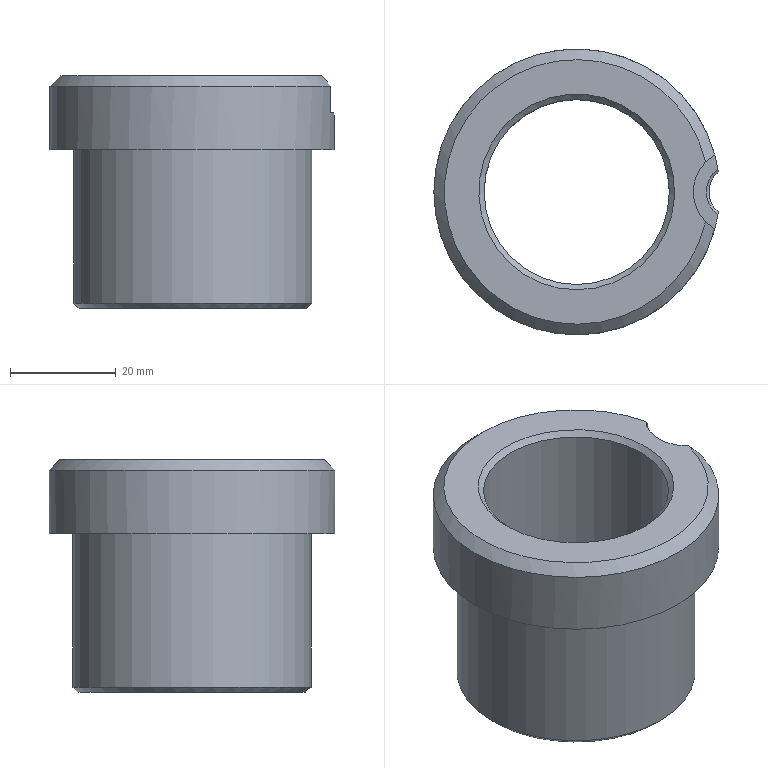Component | NX | DRILL_BUSH | 1 solid | 14 faces | box 53.73 x 54 x 44 mm | volume 36540 mm3 | cylinder 5 | cone 5 | plane 4 | commonest cylinder face diameters 45 x1 54 x1 35 x1 10 x1 16 x1
STEP:
#1=CARTESIAN_POINT('',(0.,0.,0.));
#2=DIRECTION('',(0.,0.,1.));
#3=DIRECTION('',(1.,0.,0.));
#4=AXIS2_PLACEMENT_3D('',#1,#2,#3);
#5=CARTESIAN_POINT('',(-37.,21.5,64.));
#6=VERTEX_POINT('',#5);
#7=CARTESIAN_POINT('',(-37.,-0.,64.));
#8=DIRECTION('',(0.,0.,-1.));
#9=DIRECTION('',(0.,1.,0.));
#10=AXIS2_PLACEMENT_3D('',#7,#8,#9);
#11=CIRCLE('',#10,21.5);
#12=CARTESIAN_POINT('',(-37.,-0.,64.));
#13=DIRECTION('',(0.,0.,-1.));
#14=DIRECTION('',(0.,1.,0.));
#15=AXIS2_PLACEMENT_3D('',#12,#13,#14);
#16=PLANE('',#15);
#17=CARTESIAN_POINT('',(0.,0.));
#18=DIRECTION('',(1.,0.));
#19=AXIS2_PLACEMENT_2D('',#17,#18);
#20=CIRCLE('',#19,21.5);
#21=(GEOMETRIC_REPRESENTATION_CONTEXT(2)PARAMETRIC_REPRESENTATION_CONTEXT()REPRESENTATION_CONTEXT('',''));
#22=DEFINITIONAL_REPRESENTATION('',(#20),#21);
#23=PCURVE('',#16,#22);
#24=CARTESIAN_POINT('',(-37.,-0.,65.));
#25=DIRECTION('',(0.,0.,1.));
#26=DIRECTION('',(0.,-1.,0.));
#27=AXIS2_PLACEMENT_3D('',#24,#25,#26);
#28=CONICAL_SURFACE('',#27,22.5,0.7854);
#29=CARTESIAN_POINT('',(9.425,-1.));
#30=DIRECTION('',(-1.,0.));
#31=VECTOR('',#30,1.);
#32=LINE('',#29,#31);
#33=(GEOMETRIC_REPRESENTATION_CONTEXT(2)PARAMETRIC_REPRESENTATION_CONTEXT()REPRESENTATION_CONTEXT('',''));
#34=DEFINITIONAL_REPRESENTATION('',(#32),#33);
#35=PCURVE('',#28,#34);
#36=SURFACE_CURVE('',#11,(#23,#35),.PCURVE_S1.);
#37=EDGE_CURVE('',#6,#6,#36,.T.);
#38=ORIENTED_EDGE('',*,*,#37,.T.);
#39=EDGE_LOOP('',(#38));
#40=FACE_BOUND('',#39,.T.);
#41=CARTESIAN_POINT('',(-37.,18.5,64.));
#42=VERTEX_POINT('',#41);
#43=CARTESIAN_POINT('',(-37.,-0.,64.));
#44=DIRECTION('',(0.,0.,1.));
#45=DIRECTION('',(0.,1.,0.));
#46=AXIS2_PLACEMENT_3D('',#43,#44,#45);
#47=CIRCLE('',#46,18.5);
#48=CARTESIAN_POINT('',(18.5,0.));
#49=CARTESIAN_POINT('',(18.5,-32.043));
#50=CARTESIAN_POINT('',(-9.25,-16.021));
#51=CARTESIAN_POINT('',(-37.,-0.));
#52=CARTESIAN_POINT('',(-9.25,16.021));
#53=CARTESIAN_POINT('',(18.5,32.043));
#54=CARTESIAN_POINT('',(18.5,0.));
#55=(BOUNDED_CURVE()B_SPLINE_CURVE(2,(#48,#49,#50,#51,#52,#53,#54),.UNSPECIFIED.,.T.,.F.)B_SPLINE_CURVE_WITH_KNOTS((1,2,2,2,2,1),(-2.094,0.,2.094,4.189,6.283,8.378),.UNSPECIFIED.)CURVE()GEOMETRIC_REPRESENTATION_ITEM()RATIONAL_B_SPLINE_CURVE((1.,0.5,1.,0.5,1.,0.5,1.))REPRESENTATION_ITEM(''));
#56=(GEOMETRIC_REPRESENTATION_CONTEXT(2)PARAMETRIC_REPRESENTATION_CONTEXT()REPRESENTATION_CONTEXT('',''));
#57=DEFINITIONAL_REPRESENTATION('',(#55),#56);
#58=PCURVE('',#16,#57);
#59=CARTESIAN_POINT('',(-37.,-0.,65.));
#60=DIRECTION('',(0.,0.,-1.));
#61=DIRECTION('',(0.,1.,0.));
#62=AXIS2_PLACEMENT_3D('',#59,#60,#61);
#63=CONICAL_SURFACE('',#62,17.5,0.7854);
#64=CARTESIAN_POINT('',(6.283,1.));
#65=DIRECTION('',(-1.,0.));
#66=VECTOR('',#65,1.);
#67=LINE('',#64,#66);
#68=(GEOMETRIC_REPRESENTATION_CONTEXT(2)PARAMETRIC_REPRESENTATION_CONTEXT()REPRESENTATION_CONTEXT('',''));
#69=DEFINITIONAL_REPRESENTATION('',(#67),#68);
#70=PCURVE('',#63,#69);
#71=SURFACE_CURVE('',#47,(#58,#70),.PCURVE_S1.);
#72=EDGE_CURVE('',#42,#42,#71,.T.);
#73=ORIENTED_EDGE('',*,*,#72,.T.);
#74=EDGE_LOOP('',(#73));
#75=FACE_BOUND('',#74,.T.);
#76=ADVANCED_FACE('',(#40,#75),#16,.T.);
#77=CARTESIAN_POINT('',(-37.,22.5,65.));
#78=VERTEX_POINT('',#77);
#79=CARTESIAN_POINT('',(-37.,-0.,65.));
#80=DIRECTION('',(0.,0.,1.));
#81=DIRECTION('',(0.,1.,0.));
#82=AXIS2_PLACEMENT_3D('',#79,#80,#81);
#83=CIRCLE('',#82,22.5);
#84=CARTESIAN_POINT('',(-37.,-0.,64.));
#85=DIRECTION('',(0.,0.,1.));
#86=DIRECTION('',(0.,-1.,0.));
#87=AXIS2_PLACEMENT_3D('',#84,#85,#86);
#88=CYLINDRICAL_SURFACE('',#87,22.5);
#89=CARTESIAN_POINT('',(3.142,1.));
#90=DIRECTION('',(1.,0.));
#91=VECTOR('',#90,1.);
#92=LINE('',#89,#91);
#93=(GEOMETRIC_REPRESENTATION_CONTEXT(2)PARAMETRIC_REPRESENTATION_CONTEXT()REPRESENTATION_CONTEXT('',''));
#94=DEFINITIONAL_REPRESENTATION('',(#92),#93);
#95=PCURVE('',#88,#94);
#96=CARTESIAN_POINT('',(3.142,0.));
#97=DIRECTION('',(1.,0.));
#98=VECTOR('',#97,1.);
#99=LINE('',#96,#98);
#100=(GEOMETRIC_REPRESENTATION_CONTEXT(2)PARAMETRIC_REPRESENTATION_CONTEXT()REPRESENTATION_CONTEXT('',''));
#101=DEFINITIONAL_REPRESENTATION('',(#99),#100);
#102=PCURVE('',#28,#101);
#103=SURFACE_CURVE('',#83,(#95,#102),.PCURVE_S1.);
#104=EDGE_CURVE('',#78,#78,#103,.T.);
#105=ORIENTED_EDGE('',*,*,#104,.T.);
#106=CARTESIAN_POINT('',(-37.,22.5,94.));
#107=VERTEX_POINT('',#106);
#108=CARTESIAN_POINT('',(-37.,22.5,65.));
#109=CARTESIAN_POINT('',(-37.,22.5,94.));
#110=B_SPLINE_CURVE_WITH_KNOTS('',1,(#108,#109),.UNSPECIFIED.,.F.,.F.,(2,2),(1.,30.),.PIECEWISE_BEZIER_KNOTS.);
#111=CARTESIAN_POINT('',(9.425,0.));
#112=DIRECTION('',(0.,1.));
#113=VECTOR('',#112,1.);
#114=LINE('',#111,#113);
#115=(GEOMETRIC_REPRESENTATION_CONTEXT(2)PARAMETRIC_REPRESENTATION_CONTEXT()REPRESENTATION_CONTEXT('',''));
#116=DEFINITIONAL_REPRESENTATION('',(#114),#115);
#117=PCURVE('',#88,#116);
#118=CARTESIAN_POINT('',(3.142,0.));
#119=DIRECTION('',(0.,1.));
#120=VECTOR('',#119,1.);
#121=LINE('',#118,#120);
#122=(GEOMETRIC_REPRESENTATION_CONTEXT(2)PARAMETRIC_REPRESENTATION_CONTEXT()REPRESENTATION_CONTEXT('',''));
#123=DEFINITIONAL_REPRESENTATION('',(#121),#122);
#124=PCURVE('',#88,#123);
#125=SEAM_CURVE('',#110,(#117,#124),.PCURVE_S1.);
#126=EDGE_CURVE('',#78,#107,#125,.T.);
#127=ORIENTED_EDGE('',*,*,#126,.T.);
#128=CARTESIAN_POINT('',(-37.,-0.,94.));
#129=DIRECTION('',(0.,0.,1.));
#130=DIRECTION('',(0.,1.,0.));
#131=AXIS2_PLACEMENT_3D('',#128,#129,#130);
#132=CIRCLE('',#131,22.5);
#133=CARTESIAN_POINT('',(3.142,30.));
#134=DIRECTION('',(1.,0.));
#135=VECTOR('',#134,1.);
#136=LINE('',#133,#135);
#137=(GEOMETRIC_REPRESENTATION_CONTEXT(2)PARAMETRIC_REPRESENTATION_CONTEXT()REPRESENTATION_CONTEXT('',''));
#138=DEFINITIONAL_REPRESENTATION('',(#136),#137);
#139=PCURVE('',#88,#138);
#140=CARTESIAN_POINT('',(-37.,-0.,94.));
#141=DIRECTION('',(0.,0.,-1.));
#142=DIRECTION('',(0.,1.,0.));
#143=AXIS2_PLACEMENT_3D('',#140,#141,#142);
#144=PLANE('',#143);
#145=CARTESIAN_POINT('',(22.5,0.));
#146=CARTESIAN_POINT('',(22.5,-38.971));
#147=CARTESIAN_POINT('',(-11.25,-19.486));
#148=CARTESIAN_POINT('',(-45.,-0.));
#149=CARTESIAN_POINT('',(-11.25,19.486));
#150=CARTESIAN_POINT('',(22.5,38.971));
#151=CARTESIAN_POINT('',(22.5,0.));
#152=(BOUNDED_CURVE()B_SPLINE_CURVE(2,(#145,#146,#147,#148,#149,#150,#151),.UNSPECIFIED.,.T.,.F.)B_SPLINE_CURVE_WITH_KNOTS((1,2,2,2,2,1),(-2.094,0.,2.094,4.189,6.283,8.378),.UNSPECIFIED.)CURVE()GEOMETRIC_REPRESENTATION_ITEM()RATIONAL_B_SPLINE_CURVE((1.,0.5,1.,0.5,1.,0.5,1.))REPRESENTATION_ITEM(''));
#153=(GEOMETRIC_REPRESENTATION_CONTEXT(2)PARAMETRIC_REPRESENTATION_CONTEXT()REPRESENTATION_CONTEXT('',''));
#154=DEFINITIONAL_REPRESENTATION('',(#152),#153);
#155=PCURVE('',#144,#154);
#156=SURFACE_CURVE('',#132,(#139,#155),.PCURVE_S1.);
#157=EDGE_CURVE('',#107,#107,#156,.T.);
#158=ORIENTED_EDGE('',*,*,#157,.F.);
#159=ORIENTED_EDGE('',*,*,#126,.F.);
#160=EDGE_LOOP('',(#105,#127,#158,#159));
#161=FACE_BOUND('',#160,.T.);
#162=ADVANCED_FACE('',(#161),#88,.T.);
#163=CARTESIAN_POINT('',(-37.,-18.5,108.));
#164=VERTEX_POINT('',#163);
#165=CARTESIAN_POINT('',(-37.,-0.,108.));
#166=DIRECTION('',(0.,0.,-1.));
#167=DIRECTION('',(0.,-1.,0.));
#168=AXIS2_PLACEMENT_3D('',#165,#166,#167);
#169=CIRCLE('',#168,18.5);
#170=CARTESIAN_POINT('',(-37.,-0.,108.));
#171=DIRECTION('',(0.,0.,1.));
#172=DIRECTION('',(0.,-1.,0.));
#173=AXIS2_PLACEMENT_3D('',#170,#171,#172);
#174=PLANE('',#173);
#175=CARTESIAN_POINT('',(18.5,0.));
#176=CARTESIAN_POINT('',(18.5,-32.043));
#177=CARTESIAN_POINT('',(-9.25,-16.021));
#178=CARTESIAN_POINT('',(-37.,-0.));
#179=CARTESIAN_POINT('',(-9.25,16.021));
#180=CARTESIAN_POINT('',(18.5,32.043));
#181=CARTESIAN_POINT('',(18.5,0.));
#182=(BOUNDED_CURVE()B_SPLINE_CURVE(2,(#175,#176,#177,#178,#179,#180,#181),.UNSPECIFIED.,.T.,.F.)B_SPLINE_CURVE_WITH_KNOTS((1,2,2,2,2,1),(-2.094,0.,2.094,4.189,6.283,8.378),.UNSPECIFIED.)CURVE()GEOMETRIC_REPRESENTATION_ITEM()RATIONAL_B_SPLINE_CURVE((1.,0.5,1.,0.5,1.,0.5,1.))REPRESENTATION_ITEM(''));
#183=(GEOMETRIC_REPRESENTATION_CONTEXT(2)PARAMETRIC_REPRESENTATION_CONTEXT()REPRESENTATION_CONTEXT('',''));
#184=DEFINITIONAL_REPRESENTATION('',(#182),#183);
#185=PCURVE('',#174,#184);
#186=CARTESIAN_POINT('',(-37.,-0.,108.));
#187=DIRECTION('',(0.,0.,1.));
#188=DIRECTION('',(0.,-1.,0.));
#189=AXIS2_PLACEMENT_3D('',#186,#187,#188);
#190=CONICAL_SURFACE('',#189,18.5,0.7854);
#191=CARTESIAN_POINT('',(6.283,0.));
#192=DIRECTION('',(-1.,0.));
#193=VECTOR('',#192,1.);
#194=LINE('',#191,#193);
#195=(GEOMETRIC_REPRESENTATION_CONTEXT(2)PARAMETRIC_REPRESENTATION_CONTEXT()REPRESENTATION_CONTEXT('',''));
#196=DEFINITIONAL_REPRESENTATION('',(#194),#195);
#197=PCURVE('',#190,#196);
#198=SURFACE_CURVE('',#169,(#185,#197),.PCURVE_S1.);
#199=EDGE_CURVE('',#164,#164,#198,.T.);
#200=ORIENTED_EDGE('',*,*,#199,.T.);
#201=EDGE_LOOP('',(#200));
#202=FACE_BOUND('',#201,.T.);
#203=CARTESIAN_POINT('',(-12.65,-5.664,108.));
#204=VERTEX_POINT('',#203);
#205=CARTESIAN_POINT('',(-12.65,5.664,108.));
#206=VERTEX_POINT('',#205);
#207=CARTESIAN_POINT('',(-7.,-0.,108.));
#208=DIRECTION('',(0.,0.,-1.));
#209=DIRECTION('',(0.,1.,0.));
#210=AXIS2_PLACEMENT_3D('',#207,#208,#209);
#211=CIRCLE('',#210,8.);
#212=CARTESIAN_POINT('',(-8.,30.));
#213=CARTESIAN_POINT('',(-8.,43.856));
#214=CARTESIAN_POINT('',(4.,36.928));
#215=CARTESIAN_POINT('',(16.,30.));
#216=CARTESIAN_POINT('',(4.,23.072));
#217=CARTESIAN_POINT('',(-8.,16.144));
#218=CARTESIAN_POINT('',(-8.,30.));
#219=(BOUNDED_CURVE()B_SPLINE_CURVE(2,(#212,#213,#214,#215,#216,#217,#218),.UNSPECIFIED.,.T.,.F.)B_SPLINE_CURVE_WITH_KNOTS((1,2,2,2,2,1),(-2.094,0.,2.094,4.189,6.283,8.378),.UNSPECIFIED.)CURVE()GEOMETRIC_REPRESENTATION_ITEM()RATIONAL_B_SPLINE_CURVE((1.,0.5,1.,0.5,1.,0.5,1.))REPRESENTATION_ITEM(''));
#220=(GEOMETRIC_REPRESENTATION_CONTEXT(2)PARAMETRIC_REPRESENTATION_CONTEXT()REPRESENTATION_CONTEXT('',''));
#221=DEFINITIONAL_REPRESENTATION('',(#219),#220);
#222=PCURVE('',#174,#221);
#223=CARTESIAN_POINT('',(-7.,-0.,108.));
#224=DIRECTION('',(0.,0.,-1.));
#225=DIRECTION('',(0.,1.,0.));
#226=AXIS2_PLACEMENT_3D('',#223,#224,#225);
#227=CYLINDRICAL_SURFACE('',#226,8.);
#228=CARTESIAN_POINT('',(-0.,0.));
#229=DIRECTION('',(1.,0.));
#230=VECTOR('',#229,1.);
#231=LINE('',#228,#230);
#232=(GEOMETRIC_REPRESENTATION_CONTEXT(2)PARAMETRIC_REPRESENTATION_CONTEXT()REPRESENTATION_CONTEXT('',''));
#233=DEFINITIONAL_REPRESENTATION('',(#231),#232);
#234=PCURVE('',#227,#233);
#235=SURFACE_CURVE('',#211,(#222,#234),.PCURVE_S1.);
#236=EDGE_CURVE('',#204,#206,#235,.T.);
#237=ORIENTED_EDGE('',*,*,#236,.T.);
#238=CARTESIAN_POINT('',(-37.,-0.,108.));
#239=DIRECTION('',(0.,0.,1.));
#240=DIRECTION('',(0.,-1.,0.));
#241=AXIS2_PLACEMENT_3D('',#238,#239,#240);
#242=CIRCLE('',#241,25.);
#243=CARTESIAN_POINT('',(0.,0.));
#244=DIRECTION('',(1.,0.));
#245=AXIS2_PLACEMENT_2D('',#243,#244);
#246=CIRCLE('',#245,25.);
#247=(GEOMETRIC_REPRESENTATION_CONTEXT(2)PARAMETRIC_REPRESENTATION_CONTEXT()REPRESENTATION_CONTEXT('',''));
#248=DEFINITIONAL_REPRESENTATION('',(#246),#247);
#249=PCURVE('',#174,#248);
#250=CARTESIAN_POINT('',(-37.,-0.,106.));
#251=DIRECTION('',(0.,0.,-1.));
#252=DIRECTION('',(0.,1.,0.));
#253=AXIS2_PLACEMENT_3D('',#250,#251,#252);
#254=CONICAL_SURFACE('',#253,27.,0.7854);
#255=CARTESIAN_POINT('',(9.425,-2.));
#256=DIRECTION('',(-1.,0.));
#257=VECTOR('',#256,1.);
#258=LINE('',#255,#257);
#259=(GEOMETRIC_REPRESENTATION_CONTEXT(2)PARAMETRIC_REPRESENTATION_CONTEXT()REPRESENTATION_CONTEXT('',''));
#260=DEFINITIONAL_REPRESENTATION('',(#258),#259);
#261=PCURVE('',#254,#260);
#262=SURFACE_CURVE('',#242,(#249,#261),.PCURVE_S1.);
#263=EDGE_CURVE('',#206,#204,#262,.T.);
#264=ORIENTED_EDGE('',*,*,#263,.T.);
#265=EDGE_LOOP('',(#237,#264));
#266=FACE_BOUND('',#265,.T.);
#267=ADVANCED_FACE('',(#202,#266),#174,.T.);
#268=CARTESIAN_POINT('',(-10.267,-3.785,94.));
#269=VERTEX_POINT('',#268);
#270=CARTESIAN_POINT('',(-10.267,3.785,94.));
#271=VERTEX_POINT('',#270);
#272=CARTESIAN_POINT('',(-7.,-0.,94.));
#273=DIRECTION('',(0.,0.,-1.));
#274=DIRECTION('',(0.,1.,0.));
#275=AXIS2_PLACEMENT_3D('',#272,#273,#274);
#276=CIRCLE('',#275,5.);
#277=CARTESIAN_POINT('',(0.,30.));
#278=DIRECTION('',(1.,0.));
#279=AXIS2_PLACEMENT_2D('',#277,#278);
#280=CIRCLE('',#279,5.);
#281=(GEOMETRIC_REPRESENTATION_CONTEXT(2)PARAMETRIC_REPRESENTATION_CONTEXT()REPRESENTATION_CONTEXT('',''));
#282=DEFINITIONAL_REPRESENTATION('',(#280),#281);
#283=PCURVE('',#144,#282);
#284=CARTESIAN_POINT('',(-7.,-0.,45.524));
#285=DIRECTION('',(0.,0.,-1.));
#286=DIRECTION('',(0.,1.,0.));
#287=AXIS2_PLACEMENT_3D('',#284,#285,#286);
#288=CYLINDRICAL_SURFACE('',#287,5.);
#289=CARTESIAN_POINT('',(0.,-48.476));
#290=DIRECTION('',(1.,0.));
#291=VECTOR('',#290,1.);
#292=LINE('',#289,#291);
#293=(GEOMETRIC_REPRESENTATION_CONTEXT(2)PARAMETRIC_REPRESENTATION_CONTEXT()REPRESENTATION_CONTEXT('',''));
#294=DEFINITIONAL_REPRESENTATION('',(#292),#293);
#295=PCURVE('',#288,#294);
#296=SURFACE_CURVE('',#276,(#283,#295),.PCURVE_S1.);
#297=EDGE_CURVE('',#269,#271,#296,.T.);
#298=ORIENTED_EDGE('',*,*,#297,.F.);
#299=CARTESIAN_POINT('',(-37.,-0.,94.));
#300=DIRECTION('',(0.,0.,1.));
#301=DIRECTION('',(0.,-1.,0.));
#302=AXIS2_PLACEMENT_3D('',#299,#300,#301);
#303=CIRCLE('',#302,27.);
#304=CARTESIAN_POINT('',(-27.,0.));
#305=CARTESIAN_POINT('',(-27.,46.765));
#306=CARTESIAN_POINT('',(13.5,23.383));
#307=CARTESIAN_POINT('',(54.,0.));
#308=CARTESIAN_POINT('',(13.5,-23.383));
#309=CARTESIAN_POINT('',(-27.,-46.765));
#310=CARTESIAN_POINT('',(-27.,0.));
#311=(BOUNDED_CURVE()B_SPLINE_CURVE(2,(#304,#305,#306,#307,#308,#309,#310),.UNSPECIFIED.,.T.,.F.)B_SPLINE_CURVE_WITH_KNOTS((1,2,2,2,2,1),(-2.094,0.,2.094,4.189,6.283,8.378),.UNSPECIFIED.)CURVE()GEOMETRIC_REPRESENTATION_ITEM()RATIONAL_B_SPLINE_CURVE((1.,0.5,1.,0.5,1.,0.5,1.))REPRESENTATION_ITEM(''));
#312=(GEOMETRIC_REPRESENTATION_CONTEXT(2)PARAMETRIC_REPRESENTATION_CONTEXT()REPRESENTATION_CONTEXT('',''));
#313=DEFINITIONAL_REPRESENTATION('',(#311),#312);
#314=PCURVE('',#144,#313);
#315=CARTESIAN_POINT('',(-37.,-0.,94.));
#316=DIRECTION('',(0.,0.,1.));
#317=DIRECTION('',(0.,-1.,0.));
#318=AXIS2_PLACEMENT_3D('',#315,#316,#317);
#319=CYLINDRICAL_SURFACE('',#318,27.);
#320=CARTESIAN_POINT('',(0.,0.));
#321=DIRECTION('',(1.,0.));
#322=VECTOR('',#321,1.);
#323=LINE('',#320,#322);
#324=(GEOMETRIC_REPRESENTATION_CONTEXT(2)PARAMETRIC_REPRESENTATION_CONTEXT()REPRESENTATION_CONTEXT('',''));
#325=DEFINITIONAL_REPRESENTATION('',(#323),#324);
#326=PCURVE('',#319,#325);
#327=SURFACE_CURVE('',#303,(#314,#326),.PCURVE_S1.);
#328=EDGE_CURVE('',#271,#269,#327,.T.);
#329=ORIENTED_EDGE('',*,*,#328,.F.);
#330=EDGE_LOOP('',(#298,#329));
#331=FACE_BOUND('',#330,.T.);
#332=ORIENTED_EDGE('',*,*,#157,.T.);
#333=EDGE_LOOP('',(#332));
#334=FACE_BOUND('',#333,.T.);
#335=ADVANCED_FACE('',(#331,#334),#144,.T.);
#336=CARTESIAN_POINT('',(-10.267,-3.785,100.5));
#337=VERTEX_POINT('',#336);
#338=CARTESIAN_POINT('',(-10.267,-3.785,73.262));
#339=DIRECTION('',(0.,0.,-1.));
#340=VECTOR('',#339,1.);
#341=LINE('',#338,#340);
#342=CARTESIAN_POINT('',(7.713,-20.738));
#343=DIRECTION('',(0.,-1.));
#344=VECTOR('',#343,1.);
#345=LINE('',#342,#344);
#346=(GEOMETRIC_REPRESENTATION_CONTEXT(2)PARAMETRIC_REPRESENTATION_CONTEXT()REPRESENTATION_CONTEXT('',''));
#347=DEFINITIONAL_REPRESENTATION('',(#345),#346);
#348=PCURVE('',#319,#347);
#349=CARTESIAN_POINT('',(3.854,-27.738));
#350=DIRECTION('',(0.,1.));
#351=VECTOR('',#350,1.);
#352=LINE('',#349,#351);
#353=(GEOMETRIC_REPRESENTATION_CONTEXT(2)PARAMETRIC_REPRESENTATION_CONTEXT()REPRESENTATION_CONTEXT('',''));
#354=DEFINITIONAL_REPRESENTATION('',(#352),#353);
#355=PCURVE('',#288,#354);
#356=SURFACE_CURVE('',#341,(#348,#355),.PCURVE_S1.);
#357=EDGE_CURVE('',#337,#269,#356,.T.);
#358=ORIENTED_EDGE('',*,*,#357,.F.);
#359=CARTESIAN_POINT('',(-10.354,-4.359,101.));
#360=VERTEX_POINT('',#359);
#361=CARTESIAN_POINT('',(-10.267,-3.785,100.5));
#362=CARTESIAN_POINT('',(-10.294,-3.979,100.664));
#363=CARTESIAN_POINT('',(-10.323,-4.17,100.831));
#364=CARTESIAN_POINT('',(-10.354,-4.359,101.));
#365=B_SPLINE_CURVE_WITH_KNOTS('',3,(#361,#362,#363,#364),.UNSPECIFIED.,.F.,.F.,(4,4),(0.,1.),.PIECEWISE_BEZIER_KNOTS.);
#366=CARTESIAN_POINT('',(7.713,6.5));
#367=CARTESIAN_POINT('',(7.692,7.));
#368=B_SPLINE_CURVE_WITH_KNOTS('',1,(#366,#367),.UNSPECIFIED.,.F.,.F.,(2,2),(0.,1.),.PIECEWISE_BEZIER_KNOTS.);
#369=(GEOMETRIC_REPRESENTATION_CONTEXT(2)PARAMETRIC_REPRESENTATION_CONTEXT()REPRESENTATION_CONTEXT('',''));
#370=DEFINITIONAL_REPRESENTATION('',(#368),#369);
#371=PCURVE('',#319,#370);
#372=CARTESIAN_POINT('',(-7.,-0.,100.5));
#373=DIRECTION('',(0.,0.,1.));
#374=DIRECTION('',(0.,-1.,0.));
#375=AXIS2_PLACEMENT_3D('',#372,#373,#374);
#376=CONICAL_SURFACE('',#375,5.,0.7854);
#377=CARTESIAN_POINT('',(5.571,-0.));
#378=CARTESIAN_POINT('',(5.627,0.5));
#379=B_SPLINE_CURVE_WITH_KNOTS('',1,(#377,#378),.UNSPECIFIED.,.F.,.F.,(2,2),(0.,1.),.PIECEWISE_BEZIER_KNOTS.);
#380=(GEOMETRIC_REPRESENTATION_CONTEXT(2)PARAMETRIC_REPRESENTATION_CONTEXT()REPRESENTATION_CONTEXT('',''));
#381=DEFINITIONAL_REPRESENTATION('',(#379),#380);
#382=PCURVE('',#376,#381);
#383=SURFACE_CURVE('',#365,(#371,#382),.PCURVE_S1.);
#384=EDGE_CURVE('',#337,#360,#383,.T.);
#385=ORIENTED_EDGE('',*,*,#384,.T.);
#386=CARTESIAN_POINT('',(-10.917,-6.976,101.));
#387=VERTEX_POINT('',#386);
#388=CARTESIAN_POINT('',(-37.,-0.,101.));
#389=DIRECTION('',(0.,0.,1.));
#390=DIRECTION('',(0.,1.,0.));
#391=AXIS2_PLACEMENT_3D('',#388,#389,#390);
#392=CIRCLE('',#391,27.);
#393=CARTESIAN_POINT('',(3.142,7.));
#394=DIRECTION('',(1.,0.));
#395=VECTOR('',#394,1.);
#396=LINE('',#393,#395);
#397=(GEOMETRIC_REPRESENTATION_CONTEXT(2)PARAMETRIC_REPRESENTATION_CONTEXT()REPRESENTATION_CONTEXT('',''));
#398=DEFINITIONAL_REPRESENTATION('',(#396),#397);
#399=PCURVE('',#319,#398);
#400=CARTESIAN_POINT('',(-7.,-0.,101.));
#401=DIRECTION('',(0.,0.,-1.));
#402=DIRECTION('',(0.,1.,0.));
#403=AXIS2_PLACEMENT_3D('',#400,#401,#402);
#404=PLANE('',#403);
#405=CARTESIAN_POINT('',(27.,-30.));
#406=CARTESIAN_POINT('',(27.,-76.765));
#407=CARTESIAN_POINT('',(-13.5,-53.383));
#408=CARTESIAN_POINT('',(-54.,-30.));
#409=CARTESIAN_POINT('',(-13.5,-6.617));
#410=CARTESIAN_POINT('',(27.,16.765));
#411=CARTESIAN_POINT('',(27.,-30.));
#412=(BOUNDED_CURVE()B_SPLINE_CURVE(2,(#405,#406,#407,#408,#409,#410,#411),.UNSPECIFIED.,.T.,.F.)B_SPLINE_CURVE_WITH_KNOTS((1,2,2,2,2,1),(-2.094,0.,2.094,4.189,6.283,8.378),.UNSPECIFIED.)CURVE()GEOMETRIC_REPRESENTATION_ITEM()RATIONAL_B_SPLINE_CURVE((1.,0.5,1.,0.5,1.,0.5,1.))REPRESENTATION_ITEM(''));
#413=(GEOMETRIC_REPRESENTATION_CONTEXT(2)PARAMETRIC_REPRESENTATION_CONTEXT()REPRESENTATION_CONTEXT('',''));
#414=DEFINITIONAL_REPRESENTATION('',(#412),#413);
#415=PCURVE('',#404,#414);
#416=SURFACE_CURVE('',#392,(#399,#415),.PCURVE_S1.);
#417=EDGE_CURVE('',#387,#360,#416,.T.);
#418=ORIENTED_EDGE('',*,*,#417,.F.);
#419=CARTESIAN_POINT('',(-10.917,-6.976,106.));
#420=VERTEX_POINT('',#419);
#421=CARTESIAN_POINT('',(-10.917,-6.976,104.5));
#422=DIRECTION('',(0.,0.,-1.));
#423=VECTOR('',#422,1.);
#424=LINE('',#421,#423);
#425=CARTESIAN_POINT('',(7.593,10.5));
#426=DIRECTION('',(0.,-1.));
#427=VECTOR('',#426,1.);
#428=LINE('',#425,#427);
#429=(GEOMETRIC_REPRESENTATION_CONTEXT(2)PARAMETRIC_REPRESENTATION_CONTEXT()REPRESENTATION_CONTEXT('',''));
#430=DEFINITIONAL_REPRESENTATION('',(#428),#429);
#431=PCURVE('',#319,#430);
#432=CARTESIAN_POINT('',(3.653,3.5));
#433=DIRECTION('',(0.,1.));
#434=VECTOR('',#433,1.);
#435=LINE('',#432,#434);
#436=(GEOMETRIC_REPRESENTATION_CONTEXT(2)PARAMETRIC_REPRESENTATION_CONTEXT()REPRESENTATION_CONTEXT('',''));
#437=DEFINITIONAL_REPRESENTATION('',(#435),#436);
#438=PCURVE('',#227,#437);
#439=SURFACE_CURVE('',#424,(#431,#438),.PCURVE_S1.);
#440=EDGE_CURVE('',#420,#387,#439,.T.);
#441=ORIENTED_EDGE('',*,*,#440,.F.);
#442=CARTESIAN_POINT('',(-10.917,6.976,106.));
#443=VERTEX_POINT('',#442);
#444=CARTESIAN_POINT('',(-37.,-0.,106.));
#445=DIRECTION('',(0.,0.,-1.));
#446=DIRECTION('',(0.,-1.,0.));
#447=AXIS2_PLACEMENT_3D('',#444,#445,#446);
#448=CIRCLE('',#447,27.);
#449=CARTESIAN_POINT('',(12.566,12.));
#450=DIRECTION('',(-1.,0.));
#451=VECTOR('',#450,1.);
#452=LINE('',#449,#451);
#453=(GEOMETRIC_REPRESENTATION_CONTEXT(2)PARAMETRIC_REPRESENTATION_CONTEXT()REPRESENTATION_CONTEXT('',''));
#454=DEFINITIONAL_REPRESENTATION('',(#452),#453);
#455=PCURVE('',#319,#454);
#456=CARTESIAN_POINT('',(-3.142,0.));
#457=DIRECTION('',(1.,0.));
#458=VECTOR('',#457,1.);
#459=LINE('',#456,#458);
#460=(GEOMETRIC_REPRESENTATION_CONTEXT(2)PARAMETRIC_REPRESENTATION_CONTEXT()REPRESENTATION_CONTEXT('',''));
#461=DEFINITIONAL_REPRESENTATION('',(#459),#460);
#462=PCURVE('',#254,#461);
#463=SURFACE_CURVE('',#448,(#455,#462),.PCURVE_S1.);
#464=EDGE_CURVE('',#420,#443,#463,.T.);
#465=ORIENTED_EDGE('',*,*,#464,.T.);
#466=CARTESIAN_POINT('',(-10.917,6.976,101.));
#467=VERTEX_POINT('',#466);
#468=CARTESIAN_POINT('',(-10.917,6.976,104.5));
#469=DIRECTION('',(0.,0.,1.));
#470=VECTOR('',#469,1.);
#471=LINE('',#468,#470);
#472=CARTESIAN_POINT('',(1.832,10.5));
#473=DIRECTION('',(0.,1.));
#474=VECTOR('',#473,1.);
#475=LINE('',#472,#474);
#476=(GEOMETRIC_REPRESENTATION_CONTEXT(2)PARAMETRIC_REPRESENTATION_CONTEXT()REPRESENTATION_CONTEXT('',''));
#477=DEFINITIONAL_REPRESENTATION('',(#475),#476);
#478=PCURVE('',#319,#477);
#479=CARTESIAN_POINT('',(5.772,3.5));
#480=DIRECTION('',(0.,-1.));
#481=VECTOR('',#480,1.);
#482=LINE('',#479,#481);
#483=(GEOMETRIC_REPRESENTATION_CONTEXT(2)PARAMETRIC_REPRESENTATION_CONTEXT()REPRESENTATION_CONTEXT('',''));
#484=DEFINITIONAL_REPRESENTATION('',(#482),#483);
#485=PCURVE('',#227,#484);
#486=SURFACE_CURVE('',#471,(#478,#485),.PCURVE_S1.);
#487=EDGE_CURVE('',#467,#443,#486,.T.);
#488=ORIENTED_EDGE('',*,*,#487,.F.);
#489=CARTESIAN_POINT('',(-10.354,4.359,101.));
#490=VERTEX_POINT('',#489);
#491=CARTESIAN_POINT('',(-37.,-0.,101.));
#492=DIRECTION('',(0.,0.,1.));
#493=DIRECTION('',(0.,1.,0.));
#494=AXIS2_PLACEMENT_3D('',#491,#492,#493);
#495=CIRCLE('',#494,27.);
#496=CARTESIAN_POINT('',(-3.142,7.));
#497=DIRECTION('',(1.,0.));
#498=VECTOR('',#497,1.);
#499=LINE('',#496,#498);
#500=(GEOMETRIC_REPRESENTATION_CONTEXT(2)PARAMETRIC_REPRESENTATION_CONTEXT()REPRESENTATION_CONTEXT('',''));
#501=DEFINITIONAL_REPRESENTATION('',(#499),#500);
#502=PCURVE('',#319,#501);
#503=CARTESIAN_POINT('',(27.,-30.));
#504=CARTESIAN_POINT('',(27.,-76.765));
#505=CARTESIAN_POINT('',(-13.5,-53.383));
#506=CARTESIAN_POINT('',(-54.,-30.));
#507=CARTESIAN_POINT('',(-13.5,-6.617));
#508=CARTESIAN_POINT('',(27.,16.765));
#509=CARTESIAN_POINT('',(27.,-30.));
#510=(BOUNDED_CURVE()B_SPLINE_CURVE(2,(#503,#504,#505,#506,#507,#508,#509),.UNSPECIFIED.,.T.,.F.)B_SPLINE_CURVE_WITH_KNOTS((1,2,2,2,2,1),(-2.094,0.,2.094,4.189,6.283,8.378),.UNSPECIFIED.)CURVE()GEOMETRIC_REPRESENTATION_ITEM()RATIONAL_B_SPLINE_CURVE((1.,0.5,1.,0.5,1.,0.5,1.))REPRESENTATION_ITEM(''));
#511=(GEOMETRIC_REPRESENTATION_CONTEXT(2)PARAMETRIC_REPRESENTATION_CONTEXT()REPRESENTATION_CONTEXT('',''));
#512=DEFINITIONAL_REPRESENTATION('',(#510),#511);
#513=PCURVE('',#404,#512);
#514=SURFACE_CURVE('',#495,(#502,#513),.PCURVE_S1.);
#515=EDGE_CURVE('',#490,#467,#514,.T.);
#516=ORIENTED_EDGE('',*,*,#515,.F.);
#517=CARTESIAN_POINT('',(-10.267,3.785,100.5));
#518=VERTEX_POINT('',#517);
#519=CARTESIAN_POINT('',(-10.354,4.359,101.));
#520=CARTESIAN_POINT('',(-10.323,4.17,100.831));
#521=CARTESIAN_POINT('',(-10.294,3.979,100.664));
#522=CARTESIAN_POINT('',(-10.267,3.785,100.5));
#523=B_SPLINE_CURVE_WITH_KNOTS('',3,(#519,#520,#521,#522),.UNSPECIFIED.,.F.,.F.,(4,4),(0.,1.),.PIECEWISE_BEZIER_KNOTS.);
#524=CARTESIAN_POINT('',(1.733,7.));
#525=CARTESIAN_POINT('',(1.711,6.5));
#526=B_SPLINE_CURVE_WITH_KNOTS('',1,(#524,#525),.UNSPECIFIED.,.F.,.F.,(2,2),(0.,1.),.PIECEWISE_BEZIER_KNOTS.);
#527=(GEOMETRIC_REPRESENTATION_CONTEXT(2)PARAMETRIC_REPRESENTATION_CONTEXT()REPRESENTATION_CONTEXT('',''));
#528=DEFINITIONAL_REPRESENTATION('',(#526),#527);
#529=PCURVE('',#319,#528);
#530=CARTESIAN_POINT('',(3.797,0.5));
#531=CARTESIAN_POINT('',(3.854,-0.));
#532=B_SPLINE_CURVE_WITH_KNOTS('',1,(#530,#531),.UNSPECIFIED.,.F.,.F.,(2,2),(0.,1.),.PIECEWISE_BEZIER_KNOTS.);
#533=(GEOMETRIC_REPRESENTATION_CONTEXT(2)PARAMETRIC_REPRESENTATION_CONTEXT()REPRESENTATION_CONTEXT('',''));
#534=DEFINITIONAL_REPRESENTATION('',(#532),#533);
#535=PCURVE('',#376,#534);
#536=SURFACE_CURVE('',#523,(#529,#535),.PCURVE_S1.);
#537=EDGE_CURVE('',#490,#518,#536,.T.);
#538=ORIENTED_EDGE('',*,*,#537,.T.);
#539=CARTESIAN_POINT('',(-10.267,3.785,73.262));
#540=DIRECTION('',(0.,0.,1.));
#541=VECTOR('',#540,1.);
#542=LINE('',#539,#541);
#543=CARTESIAN_POINT('',(1.711,-20.738));
#544=DIRECTION('',(0.,1.));
#545=VECTOR('',#544,1.);
#546=LINE('',#543,#545);
#547=(GEOMETRIC_REPRESENTATION_CONTEXT(2)PARAMETRIC_REPRESENTATION_CONTEXT()REPRESENTATION_CONTEXT('',''));
#548=DEFINITIONAL_REPRESENTATION('',(#546),#547);
#549=PCURVE('',#319,#548);
#550=CARTESIAN_POINT('',(5.571,-27.738));
#551=DIRECTION('',(0.,-1.));
#552=VECTOR('',#551,1.);
#553=LINE('',#550,#552);
#554=(GEOMETRIC_REPRESENTATION_CONTEXT(2)PARAMETRIC_REPRESENTATION_CONTEXT()REPRESENTATION_CONTEXT('',''));
#555=DEFINITIONAL_REPRESENTATION('',(#553),#554);
#556=PCURVE('',#288,#555);
#557=SURFACE_CURVE('',#542,(#549,#556),.PCURVE_S1.);
#558=EDGE_CURVE('',#271,#518,#557,.T.);
#559=ORIENTED_EDGE('',*,*,#558,.F.);
#560=ORIENTED_EDGE('',*,*,#328,.T.);
#561=EDGE_LOOP('',(#358,#385,#418,#441,#465,#488,#516,#538,#559,#560));
#562=FACE_BOUND('',#561,.T.);
#563=ADVANCED_FACE('',(#562),#319,.T.);
#564=CARTESIAN_POINT('',(-37.,17.5,65.));
#565=VERTEX_POINT('',#564);
#566=CARTESIAN_POINT('',(-37.,-0.,65.));
#567=DIRECTION('',(0.,0.,-1.));
#568=DIRECTION('',(0.,1.,0.));
#569=AXIS2_PLACEMENT_3D('',#566,#567,#568);
#570=CIRCLE('',#569,17.5);
#571=CARTESIAN_POINT('',(-37.,-0.,108.));
#572=DIRECTION('',(0.,0.,-1.));
#573=DIRECTION('',(0.,1.,0.));
#574=AXIS2_PLACEMENT_3D('',#571,#572,#573);
#575=CYLINDRICAL_SURFACE('',#574,17.5);
#576=CARTESIAN_POINT('',(0.,43.));
#577=DIRECTION('',(1.,0.));
#578=VECTOR('',#577,1.);
#579=LINE('',#576,#578);
#580=(GEOMETRIC_REPRESENTATION_CONTEXT(2)PARAMETRIC_REPRESENTATION_CONTEXT()REPRESENTATION_CONTEXT('',''));
#581=DEFINITIONAL_REPRESENTATION('',(#579),#580);
#582=PCURVE('',#575,#581);
#583=CARTESIAN_POINT('',(0.,0.));
#584=DIRECTION('',(1.,0.));
#585=VECTOR('',#584,1.);
#586=LINE('',#583,#585);
#587=(GEOMETRIC_REPRESENTATION_CONTEXT(2)PARAMETRIC_REPRESENTATION_CONTEXT()REPRESENTATION_CONTEXT('',''));
#588=DEFINITIONAL_REPRESENTATION('',(#586),#587);
#589=PCURVE('',#63,#588);
#590=SURFACE_CURVE('',#570,(#582,#589),.PCURVE_S1.);
#591=EDGE_CURVE('',#565,#565,#590,.T.);
#592=ORIENTED_EDGE('',*,*,#591,.F.);
#593=CARTESIAN_POINT('',(-37.,17.5,107.));
#594=VERTEX_POINT('',#593);
#595=CARTESIAN_POINT('',(-37.,17.5,107.));
#596=CARTESIAN_POINT('',(-37.,17.5,65.));
#597=B_SPLINE_CURVE_WITH_KNOTS('',1,(#595,#596),.UNSPECIFIED.,.F.,.F.,(2,2),(1.,43.),.PIECEWISE_BEZIER_KNOTS.);
#598=CARTESIAN_POINT('',(0.,0.));
#599=DIRECTION('',(0.,1.));
#600=VECTOR('',#599,1.);
#601=LINE('',#598,#600);
#602=(GEOMETRIC_REPRESENTATION_CONTEXT(2)PARAMETRIC_REPRESENTATION_CONTEXT()REPRESENTATION_CONTEXT('',''));
#603=DEFINITIONAL_REPRESENTATION('',(#601),#602);
#604=PCURVE('',#575,#603);
#605=CARTESIAN_POINT('',(6.283,0.));
#606=DIRECTION('',(0.,1.));
#607=VECTOR('',#606,1.);
#608=LINE('',#605,#607);
#609=(GEOMETRIC_REPRESENTATION_CONTEXT(2)PARAMETRIC_REPRESENTATION_CONTEXT()REPRESENTATION_CONTEXT('',''));
#610=DEFINITIONAL_REPRESENTATION('',(#608),#609);
#611=PCURVE('',#575,#610);
#612=SEAM_CURVE('',#597,(#604,#611),.PCURVE_S1.);
#613=EDGE_CURVE('',#594,#565,#612,.T.);
#614=ORIENTED_EDGE('',*,*,#613,.F.);
#615=CARTESIAN_POINT('',(-37.,-17.5,107.));
#616=VERTEX_POINT('',#615);
#617=CARTESIAN_POINT('',(-37.,-0.,107.));
#618=DIRECTION('',(0.,0.,1.));
#619=DIRECTION('',(0.,-1.,0.));
#620=AXIS2_PLACEMENT_3D('',#617,#618,#619);
#621=CIRCLE('',#620,17.5);
#622=CARTESIAN_POINT('',(3.142,1.));
#623=DIRECTION('',(-1.,0.));
#624=VECTOR('',#623,1.);
#625=LINE('',#622,#624);
#626=(GEOMETRIC_REPRESENTATION_CONTEXT(2)PARAMETRIC_REPRESENTATION_CONTEXT()REPRESENTATION_CONTEXT('',''));
#627=DEFINITIONAL_REPRESENTATION('',(#625),#626);
#628=PCURVE('',#575,#627);
#629=CARTESIAN_POINT('',(0.,-1.));
#630=DIRECTION('',(1.,0.));
#631=VECTOR('',#630,1.);
#632=LINE('',#629,#631);
#633=(GEOMETRIC_REPRESENTATION_CONTEXT(2)PARAMETRIC_REPRESENTATION_CONTEXT()REPRESENTATION_CONTEXT('',''));
#634=DEFINITIONAL_REPRESENTATION('',(#632),#633);
#635=PCURVE('',#190,#634);
#636=SURFACE_CURVE('',#621,(#628,#635),.PCURVE_S1.);
#637=EDGE_CURVE('',#616,#594,#636,.T.);
#638=ORIENTED_EDGE('',*,*,#637,.F.);
#639=CARTESIAN_POINT('',(-37.,-0.,107.));
#640=DIRECTION('',(0.,0.,1.));
#641=DIRECTION('',(0.,-1.,0.));
#642=AXIS2_PLACEMENT_3D('',#639,#640,#641);
#643=CIRCLE('',#642,17.5);
#644=CARTESIAN_POINT('',(9.425,1.));
#645=DIRECTION('',(-1.,0.));
#646=VECTOR('',#645,1.);
#647=LINE('',#644,#646);
#648=(GEOMETRIC_REPRESENTATION_CONTEXT(2)PARAMETRIC_REPRESENTATION_CONTEXT()REPRESENTATION_CONTEXT('',''));
#649=DEFINITIONAL_REPRESENTATION('',(#647),#648);
#650=PCURVE('',#575,#649);
#651=CARTESIAN_POINT('',(0.,-1.));
#652=DIRECTION('',(1.,0.));
#653=VECTOR('',#652,1.);
#654=LINE('',#651,#653);
#655=(GEOMETRIC_REPRESENTATION_CONTEXT(2)PARAMETRIC_REPRESENTATION_CONTEXT()REPRESENTATION_CONTEXT('',''));
#656=DEFINITIONAL_REPRESENTATION('',(#654),#655);
#657=PCURVE('',#190,#656);
#658=SURFACE_CURVE('',#643,(#650,#657),.PCURVE_S1.);
#659=EDGE_CURVE('',#594,#616,#658,.T.);
#660=ORIENTED_EDGE('',*,*,#659,.F.);
#661=ORIENTED_EDGE('',*,*,#613,.T.);
#662=EDGE_LOOP('',(#592,#614,#638,#660,#661));
#663=FACE_BOUND('',#662,.F.);
#664=ADVANCED_FACE('',(#663),#575,.F.);
#665=ORIENTED_EDGE('',*,*,#297,.F.);
#666=ORIENTED_EDGE('',*,*,#357,.F.);
#667=CARTESIAN_POINT('',(-7.,-0.,100.5));
#668=DIRECTION('',(0.,0.,1.));
#669=DIRECTION('',(0.,1.,0.));
#670=AXIS2_PLACEMENT_3D('',#667,#668,#669);
#671=CIRCLE('',#670,5.);
#672=CARTESIAN_POINT('',(6.283,-54.976));
#673=DIRECTION('',(-1.,0.));
#674=VECTOR('',#673,1.);
#675=LINE('',#672,#674);
#676=(GEOMETRIC_REPRESENTATION_CONTEXT(2)PARAMETRIC_REPRESENTATION_CONTEXT()REPRESENTATION_CONTEXT('',''));
#677=DEFINITIONAL_REPRESENTATION('',(#675),#676);
#678=PCURVE('',#288,#677);
#679=CARTESIAN_POINT('',(3.142,0.));
#680=DIRECTION('',(1.,0.));
#681=VECTOR('',#680,1.);
#682=LINE('',#679,#681);
#683=(GEOMETRIC_REPRESENTATION_CONTEXT(2)PARAMETRIC_REPRESENTATION_CONTEXT()REPRESENTATION_CONTEXT('',''));
#684=DEFINITIONAL_REPRESENTATION('',(#682),#683);
#685=PCURVE('',#376,#684);
#686=SURFACE_CURVE('',#671,(#678,#685),.PCURVE_S1.);
#687=EDGE_CURVE('',#518,#337,#686,.T.);
#688=ORIENTED_EDGE('',*,*,#687,.F.);
#689=ORIENTED_EDGE('',*,*,#558,.F.);
#690=EDGE_LOOP('',(#665,#666,#688,#689));
#691=FACE_BOUND('',#690,.F.);
#692=ADVANCED_FACE('',(#691),#288,.F.);
#693=ORIENTED_EDGE('',*,*,#417,.T.);
#694=CARTESIAN_POINT('',(-7.,-0.,101.));
#695=DIRECTION('',(0.,0.,-1.));
#696=DIRECTION('',(0.,1.,0.));
#697=AXIS2_PLACEMENT_3D('',#694,#695,#696);
#698=CIRCLE('',#697,5.5);
#699=CARTESIAN_POINT('',(0.,0.));
#700=DIRECTION('',(1.,0.));
#701=AXIS2_PLACEMENT_2D('',#699,#700);
#702=CIRCLE('',#701,5.5);
#703=(GEOMETRIC_REPRESENTATION_CONTEXT(2)PARAMETRIC_REPRESENTATION_CONTEXT()REPRESENTATION_CONTEXT('',''));
#704=DEFINITIONAL_REPRESENTATION('',(#702),#703);
#705=PCURVE('',#404,#704);
#706=CARTESIAN_POINT('',(9.425,0.5));
#707=DIRECTION('',(-1.,0.));
#708=VECTOR('',#707,1.);
#709=LINE('',#706,#708);
#710=(GEOMETRIC_REPRESENTATION_CONTEXT(2)PARAMETRIC_REPRESENTATION_CONTEXT()REPRESENTATION_CONTEXT('',''));
#711=DEFINITIONAL_REPRESENTATION('',(#709),#710);
#712=PCURVE('',#376,#711);
#713=SURFACE_CURVE('',#698,(#705,#712),.PCURVE_S1.);
#714=EDGE_CURVE('',#360,#490,#713,.T.);
#715=ORIENTED_EDGE('',*,*,#714,.T.);
#716=ORIENTED_EDGE('',*,*,#515,.T.);
#717=CARTESIAN_POINT('',(-7.,-0.,101.));
#718=DIRECTION('',(0.,0.,1.));
#719=DIRECTION('',(0.,1.,0.));
#720=AXIS2_PLACEMENT_3D('',#717,#718,#719);
#721=CIRCLE('',#720,8.);
#722=CARTESIAN_POINT('',(8.,0.));
#723=CARTESIAN_POINT('',(8.,-13.856));
#724=CARTESIAN_POINT('',(-4.,-6.928));
#725=CARTESIAN_POINT('',(-16.,-0.));
#726=CARTESIAN_POINT('',(-4.,6.928));
#727=CARTESIAN_POINT('',(8.,13.856));
#728=CARTESIAN_POINT('',(8.,0.));
#729=(BOUNDED_CURVE()B_SPLINE_CURVE(2,(#722,#723,#724,#725,#726,#727,#728),.UNSPECIFIED.,.T.,.F.)B_SPLINE_CURVE_WITH_KNOTS((1,2,2,2,2,1),(-2.094,0.,2.094,4.189,6.283,8.378),.UNSPECIFIED.)CURVE()GEOMETRIC_REPRESENTATION_ITEM()RATIONAL_B_SPLINE_CURVE((1.,0.5,1.,0.5,1.,0.5,1.))REPRESENTATION_ITEM(''));
#730=(GEOMETRIC_REPRESENTATION_CONTEXT(2)PARAMETRIC_REPRESENTATION_CONTEXT()REPRESENTATION_CONTEXT('',''));
#731=DEFINITIONAL_REPRESENTATION('',(#729),#730);
#732=PCURVE('',#404,#731);
#733=CARTESIAN_POINT('',(6.283,7.));
#734=DIRECTION('',(-1.,0.));
#735=VECTOR('',#734,1.);
#736=LINE('',#733,#735);
#737=(GEOMETRIC_REPRESENTATION_CONTEXT(2)PARAMETRIC_REPRESENTATION_CONTEXT()REPRESENTATION_CONTEXT('',''));
#738=DEFINITIONAL_REPRESENTATION('',(#736),#737);
#739=PCURVE('',#227,#738);
#740=SURFACE_CURVE('',#721,(#732,#739),.PCURVE_S1.);
#741=EDGE_CURVE('',#467,#387,#740,.T.);
#742=ORIENTED_EDGE('',*,*,#741,.T.);
#743=EDGE_LOOP('',(#693,#715,#716,#742));
#744=FACE_BOUND('',#743,.T.);
#745=ADVANCED_FACE('',(#744),#404,.F.);
#746=ORIENTED_EDGE('',*,*,#741,.T.);
#747=ORIENTED_EDGE('',*,*,#440,.F.);
#748=CARTESIAN_POINT('',(-12.65,-5.664,108.));
#749=CARTESIAN_POINT('',(-12.116,-6.197,107.359));
#750=CARTESIAN_POINT('',(-11.537,-6.628,106.689));
#751=CARTESIAN_POINT('',(-10.917,-6.976,106.));
#752=B_SPLINE_CURVE_WITH_KNOTS('',3,(#748,#749,#750,#751),.UNSPECIFIED.,.F.,.F.,(4,4),(0.,1.),.PIECEWISE_BEZIER_KNOTS.);
#753=CARTESIAN_POINT('',(3.926,0.));
#754=CARTESIAN_POINT('',(3.653,2.));
#755=B_SPLINE_CURVE_WITH_KNOTS('',1,(#753,#754),.UNSPECIFIED.,.F.,.F.,(2,2),(0.,1.),.PIECEWISE_BEZIER_KNOTS.);
#756=(GEOMETRIC_REPRESENTATION_CONTEXT(2)PARAMETRIC_REPRESENTATION_CONTEXT()REPRESENTATION_CONTEXT('',''));
#757=DEFINITIONAL_REPRESENTATION('',(#755),#756);
#758=PCURVE('',#227,#757);
#759=CARTESIAN_POINT('',(1.799,-2.));
#760=CARTESIAN_POINT('',(1.8,-1.971));
#761=CARTESIAN_POINT('',(1.801,-1.912));
#762=CARTESIAN_POINT('',(1.804,-1.824));
#763=CARTESIAN_POINT('',(1.806,-1.736));
#764=CARTESIAN_POINT('',(1.807,-1.647));
#765=CARTESIAN_POINT('',(1.809,-1.558));
#766=CARTESIAN_POINT('',(1.811,-1.469));
#767=CARTESIAN_POINT('',(1.813,-1.379));
#768=CARTESIAN_POINT('',(1.815,-1.289));
#769=CARTESIAN_POINT('',(1.816,-1.199));
#770=CARTESIAN_POINT('',(1.818,-1.109));
#771=CARTESIAN_POINT('',(1.819,-1.018));
#772=CARTESIAN_POINT('',(1.821,-0.9266));
#773=CARTESIAN_POINT('',(1.822,-0.8351));
#774=CARTESIAN_POINT('',(1.823,-0.7434));
#775=CARTESIAN_POINT('',(1.825,-0.6514));
#776=CARTESIAN_POINT('',(1.826,-0.5591));
#777=CARTESIAN_POINT('',(1.827,-0.4666));
#778=CARTESIAN_POINT('',(1.828,-0.3738));
#779=CARTESIAN_POINT('',(1.829,-0.2807));
#780=CARTESIAN_POINT('',(1.83,-0.1874));
#781=CARTESIAN_POINT('',(1.831,-0.09384));
#782=CARTESIAN_POINT('',(1.832,-0.03131));
#783=CARTESIAN_POINT('',(1.832,0.));
#784=B_SPLINE_CURVE_WITH_KNOTS('',3,(#759,#760,#761,#762,#763,#764,#765,#766,#767,#768,#769,#770,#771,#772,#773,#774,#775,#776,#777,#778,#779,#780,#781,#782,#783),.UNSPECIFIED.,.F.,.F.,(4,1,1,1,1,1,1,1,1,1,1,1,1,1,1,1,1,1,1,1,1,1,4),(0.,0.04545,0.09091,0.1364,0.1818,0.2273,0.2727,0.3182,0.3636,0.4091,0.4545,0.5,0.5455,0.5909,0.6364,0.6818,0.7273,0.7727,0.8182,0.8636,0.9091,0.9545,1.),.QUASI_UNIFORM_KNOTS.);
#785=(GEOMETRIC_REPRESENTATION_CONTEXT(2)PARAMETRIC_REPRESENTATION_CONTEXT()REPRESENTATION_CONTEXT('',''));
#786=DEFINITIONAL_REPRESENTATION('',(#784),#785);
#787=PCURVE('',#254,#786);
#788=SURFACE_CURVE('',#752,(#758,#787),.PCURVE_S1.);
#789=EDGE_CURVE('',#204,#420,#788,.T.);
#790=ORIENTED_EDGE('',*,*,#789,.F.);
#791=ORIENTED_EDGE('',*,*,#236,.T.);
#792=CARTESIAN_POINT('',(-10.917,6.976,106.));
#793=CARTESIAN_POINT('',(-11.537,6.628,106.689));
#794=CARTESIAN_POINT('',(-12.116,6.197,107.359));
#795=CARTESIAN_POINT('',(-12.65,5.664,108.));
#796=B_SPLINE_CURVE_WITH_KNOTS('',3,(#792,#793,#794,#795),.UNSPECIFIED.,.F.,.F.,(4,4),(0.,1.),.PIECEWISE_BEZIER_KNOTS.);
#797=CARTESIAN_POINT('',(5.772,2.));
#798=CARTESIAN_POINT('',(5.499,0.));
#799=B_SPLINE_CURVE_WITH_KNOTS('',1,(#797,#798),.UNSPECIFIED.,.F.,.F.,(2,2),(0.,1.),.PIECEWISE_BEZIER_KNOTS.);
#800=(GEOMETRIC_REPRESENTATION_CONTEXT(2)PARAMETRIC_REPRESENTATION_CONTEXT()REPRESENTATION_CONTEXT('',''));
#801=DEFINITIONAL_REPRESENTATION('',(#799),#800);
#802=PCURVE('',#227,#801);
#803=CARTESIAN_POINT('',(7.593,0.));
#804=CARTESIAN_POINT('',(7.593,-0.03131));
#805=CARTESIAN_POINT('',(7.594,-0.09384));
#806=CARTESIAN_POINT('',(7.595,-0.1874));
#807=CARTESIAN_POINT('',(7.596,-0.2807));
#808=CARTESIAN_POINT('',(7.597,-0.3738));
#809=CARTESIAN_POINT('',(7.598,-0.4666));
#810=CARTESIAN_POINT('',(7.599,-0.5591));
#811=CARTESIAN_POINT('',(7.6,-0.6514));
#812=CARTESIAN_POINT('',(7.601,-0.7434));
#813=CARTESIAN_POINT('',(7.603,-0.8351));
#814=CARTESIAN_POINT('',(7.604,-0.9266));
#815=CARTESIAN_POINT('',(7.606,-1.018));
#816=CARTESIAN_POINT('',(7.607,-1.109));
#817=CARTESIAN_POINT('',(7.609,-1.199));
#818=CARTESIAN_POINT('',(7.61,-1.289));
#819=CARTESIAN_POINT('',(7.612,-1.379));
#820=CARTESIAN_POINT('',(7.614,-1.469));
#821=CARTESIAN_POINT('',(7.615,-1.558));
#822=CARTESIAN_POINT('',(7.617,-1.647));
#823=CARTESIAN_POINT('',(7.619,-1.736));
#824=CARTESIAN_POINT('',(7.621,-1.824));
#825=CARTESIAN_POINT('',(7.623,-1.912));
#826=CARTESIAN_POINT('',(7.625,-1.971));
#827=CARTESIAN_POINT('',(7.625,-2.));
#828=B_SPLINE_CURVE_WITH_KNOTS('',3,(#803,#804,#805,#806,#807,#808,#809,#810,#811,#812,#813,#814,#815,#816,#817,#818,#819,#820,#821,#822,#823,#824,#825,#826,#827),.UNSPECIFIED.,.F.,.F.,(4,1,1,1,1,1,1,1,1,1,1,1,1,1,1,1,1,1,1,1,1,1,4),(0.,0.04545,0.09091,0.1364,0.1818,0.2273,0.2727,0.3182,0.3636,0.4091,0.4545,0.5,0.5455,0.5909,0.6364,0.6818,0.7273,0.7727,0.8182,0.8636,0.9091,0.9545,1.),.QUASI_UNIFORM_KNOTS.);
#829=(GEOMETRIC_REPRESENTATION_CONTEXT(2)PARAMETRIC_REPRESENTATION_CONTEXT()REPRESENTATION_CONTEXT('',''));
#830=DEFINITIONAL_REPRESENTATION('',(#828),#829);
#831=PCURVE('',#254,#830);
#832=SURFACE_CURVE('',#796,(#802,#831),.PCURVE_S1.);
#833=EDGE_CURVE('',#443,#206,#832,.T.);
#834=ORIENTED_EDGE('',*,*,#833,.F.);
#835=ORIENTED_EDGE('',*,*,#487,.F.);
#836=EDGE_LOOP('',(#746,#747,#790,#791,#834,#835));
#837=FACE_BOUND('',#836,.F.);
#838=ADVANCED_FACE('',(#837),#227,.F.);
#839=ORIENTED_EDGE('',*,*,#789,.F.);
#840=ORIENTED_EDGE('',*,*,#263,.F.);
#841=ORIENTED_EDGE('',*,*,#833,.F.);
#842=ORIENTED_EDGE('',*,*,#464,.F.);
#843=EDGE_LOOP('',(#839,#840,#841,#842));
#844=FACE_BOUND('',#843,.T.);
#845=ADVANCED_FACE('',(#844),#254,.T.);
#846=ORIENTED_EDGE('',*,*,#37,.F.);
#847=CARTESIAN_POINT('',(-37.,21.5,64.));
#848=CARTESIAN_POINT('',(-37.,22.5,65.));
#849=B_SPLINE_CURVE_WITH_KNOTS('',1,(#847,#848),.UNSPECIFIED.,.F.,.F.,(2,2),(-1.414,0.),.PIECEWISE_BEZIER_KNOTS.);
#850=CARTESIAN_POINT('',(9.425,0.));
#851=DIRECTION('',(0.,1.));
#852=VECTOR('',#851,1.);
#853=LINE('',#850,#852);
#854=(GEOMETRIC_REPRESENTATION_CONTEXT(2)PARAMETRIC_REPRESENTATION_CONTEXT()REPRESENTATION_CONTEXT('',''));
#855=DEFINITIONAL_REPRESENTATION('',(#853),#854);
#856=PCURVE('',#28,#855);
#857=CARTESIAN_POINT('',(3.142,0.));
#858=DIRECTION('',(0.,1.));
#859=VECTOR('',#858,1.);
#860=LINE('',#857,#859);
#861=(GEOMETRIC_REPRESENTATION_CONTEXT(2)PARAMETRIC_REPRESENTATION_CONTEXT()REPRESENTATION_CONTEXT('',''));
#862=DEFINITIONAL_REPRESENTATION('',(#860),#861);
#863=PCURVE('',#28,#862);
#864=SEAM_CURVE('',#849,(#856,#863),.PCURVE_S1.);
#865=EDGE_CURVE('',#6,#78,#864,.T.);
#866=ORIENTED_EDGE('',*,*,#865,.T.);
#867=ORIENTED_EDGE('',*,*,#104,.F.);
#868=ORIENTED_EDGE('',*,*,#865,.F.);
#869=EDGE_LOOP('',(#846,#866,#867,#868));
#870=FACE_BOUND('',#869,.T.);
#871=ADVANCED_FACE('',(#870),#28,.T.);
#872=ORIENTED_EDGE('',*,*,#72,.T.);
#873=CARTESIAN_POINT('',(-37.,17.5,65.));
#874=CARTESIAN_POINT('',(-37.,18.5,64.));
#875=B_SPLINE_CURVE_WITH_KNOTS('',1,(#873,#874),.UNSPECIFIED.,.F.,.F.,(2,2),(0.,1.414),.PIECEWISE_BEZIER_KNOTS.);
#876=CARTESIAN_POINT('',(0.,0.));
#877=DIRECTION('',(0.,1.));
#878=VECTOR('',#877,1.);
#879=LINE('',#876,#878);
#880=(GEOMETRIC_REPRESENTATION_CONTEXT(2)PARAMETRIC_REPRESENTATION_CONTEXT()REPRESENTATION_CONTEXT('',''));
#881=DEFINITIONAL_REPRESENTATION('',(#879),#880);
#882=PCURVE('',#63,#881);
#883=CARTESIAN_POINT('',(6.283,0.));
#884=DIRECTION('',(0.,1.));
#885=VECTOR('',#884,1.);
#886=LINE('',#883,#885);
#887=(GEOMETRIC_REPRESENTATION_CONTEXT(2)PARAMETRIC_REPRESENTATION_CONTEXT()REPRESENTATION_CONTEXT('',''));
#888=DEFINITIONAL_REPRESENTATION('',(#886),#887);
#889=PCURVE('',#63,#888);
#890=SEAM_CURVE('',#875,(#882,#889),.PCURVE_S1.);
#891=EDGE_CURVE('',#565,#42,#890,.T.);
#892=ORIENTED_EDGE('',*,*,#891,.F.);
#893=ORIENTED_EDGE('',*,*,#591,.T.);
#894=ORIENTED_EDGE('',*,*,#891,.T.);
#895=EDGE_LOOP('',(#872,#892,#893,#894));
#896=FACE_BOUND('',#895,.F.);
#897=ADVANCED_FACE('',(#896),#63,.F.);
#898=ORIENTED_EDGE('',*,*,#659,.T.);
#899=CARTESIAN_POINT('',(-37.,-17.5,107.));
#900=CARTESIAN_POINT('',(-37.,-18.5,108.));
#901=B_SPLINE_CURVE_WITH_KNOTS('',1,(#899,#900),.UNSPECIFIED.,.F.,.F.,(2,2),(-1.414,0.),.PIECEWISE_BEZIER_KNOTS.);
#902=CARTESIAN_POINT('',(6.283,0.));
#903=DIRECTION('',(0.,1.));
#904=VECTOR('',#903,1.);
#905=LINE('',#902,#904);
#906=(GEOMETRIC_REPRESENTATION_CONTEXT(2)PARAMETRIC_REPRESENTATION_CONTEXT()REPRESENTATION_CONTEXT('',''));
#907=DEFINITIONAL_REPRESENTATION('',(#905),#906);
#908=PCURVE('',#190,#907);
#909=CARTESIAN_POINT('',(0.,0.));
#910=DIRECTION('',(0.,1.));
#911=VECTOR('',#910,1.);
#912=LINE('',#909,#911);
#913=(GEOMETRIC_REPRESENTATION_CONTEXT(2)PARAMETRIC_REPRESENTATION_CONTEXT()REPRESENTATION_CONTEXT('',''));
#914=DEFINITIONAL_REPRESENTATION('',(#912),#913);
#915=PCURVE('',#190,#914);
#916=SEAM_CURVE('',#901,(#908,#915),.PCURVE_S1.);
#917=EDGE_CURVE('',#616,#164,#916,.T.);
#918=ORIENTED_EDGE('',*,*,#917,.T.);
#919=ORIENTED_EDGE('',*,*,#199,.T.);
#920=ORIENTED_EDGE('',*,*,#917,.F.);
#921=ORIENTED_EDGE('',*,*,#637,.T.);
#922=EDGE_LOOP('',(#898,#918,#919,#920,#921));
#923=FACE_BOUND('',#922,.F.);
#924=ADVANCED_FACE('',(#923),#190,.F.);
#925=ORIENTED_EDGE('',*,*,#687,.T.);
#926=ORIENTED_EDGE('',*,*,#384,.T.);
#927=ORIENTED_EDGE('',*,*,#714,.T.);
#928=ORIENTED_EDGE('',*,*,#537,.T.);
#929=EDGE_LOOP('',(#925,#926,#927,#928));
#930=FACE_BOUND('',#929,.F.);
#931=ADVANCED_FACE('',(#930),#376,.F.);
#932=CLOSED_SHELL('',(#76,#162,#267,#335,#563,#664,#692,#745,#838,#845,#871,#897,#924,#931));
#933=MANIFOLD_SOLID_BREP('',#932);
#934=(LENGTH_UNIT()NAMED_UNIT(*)SI_UNIT(.MILLI.,.METRE.));
#935=UNCERTAINTY_MEASURE_WITH_UNIT(LENGTH_MEASURE(0.005),#934,'','');
#936=(NAMED_UNIT(*)PLANE_ANGLE_UNIT()SI_UNIT($,.RADIAN.));
#937=(NAMED_UNIT(*)SI_UNIT($,.STERADIAN.)SOLID_ANGLE_UNIT());
#938=(GEOMETRIC_REPRESENTATION_CONTEXT(3)GLOBAL_UNCERTAINTY_ASSIGNED_CONTEXT((#935))GLOBAL_UNIT_ASSIGNED_CONTEXT((#934,#936,#937))REPRESENTATION_CONTEXT('',''));
#939=ADVANCED_BREP_SHAPE_REPRESENTATION('',(#4,#933),#938);